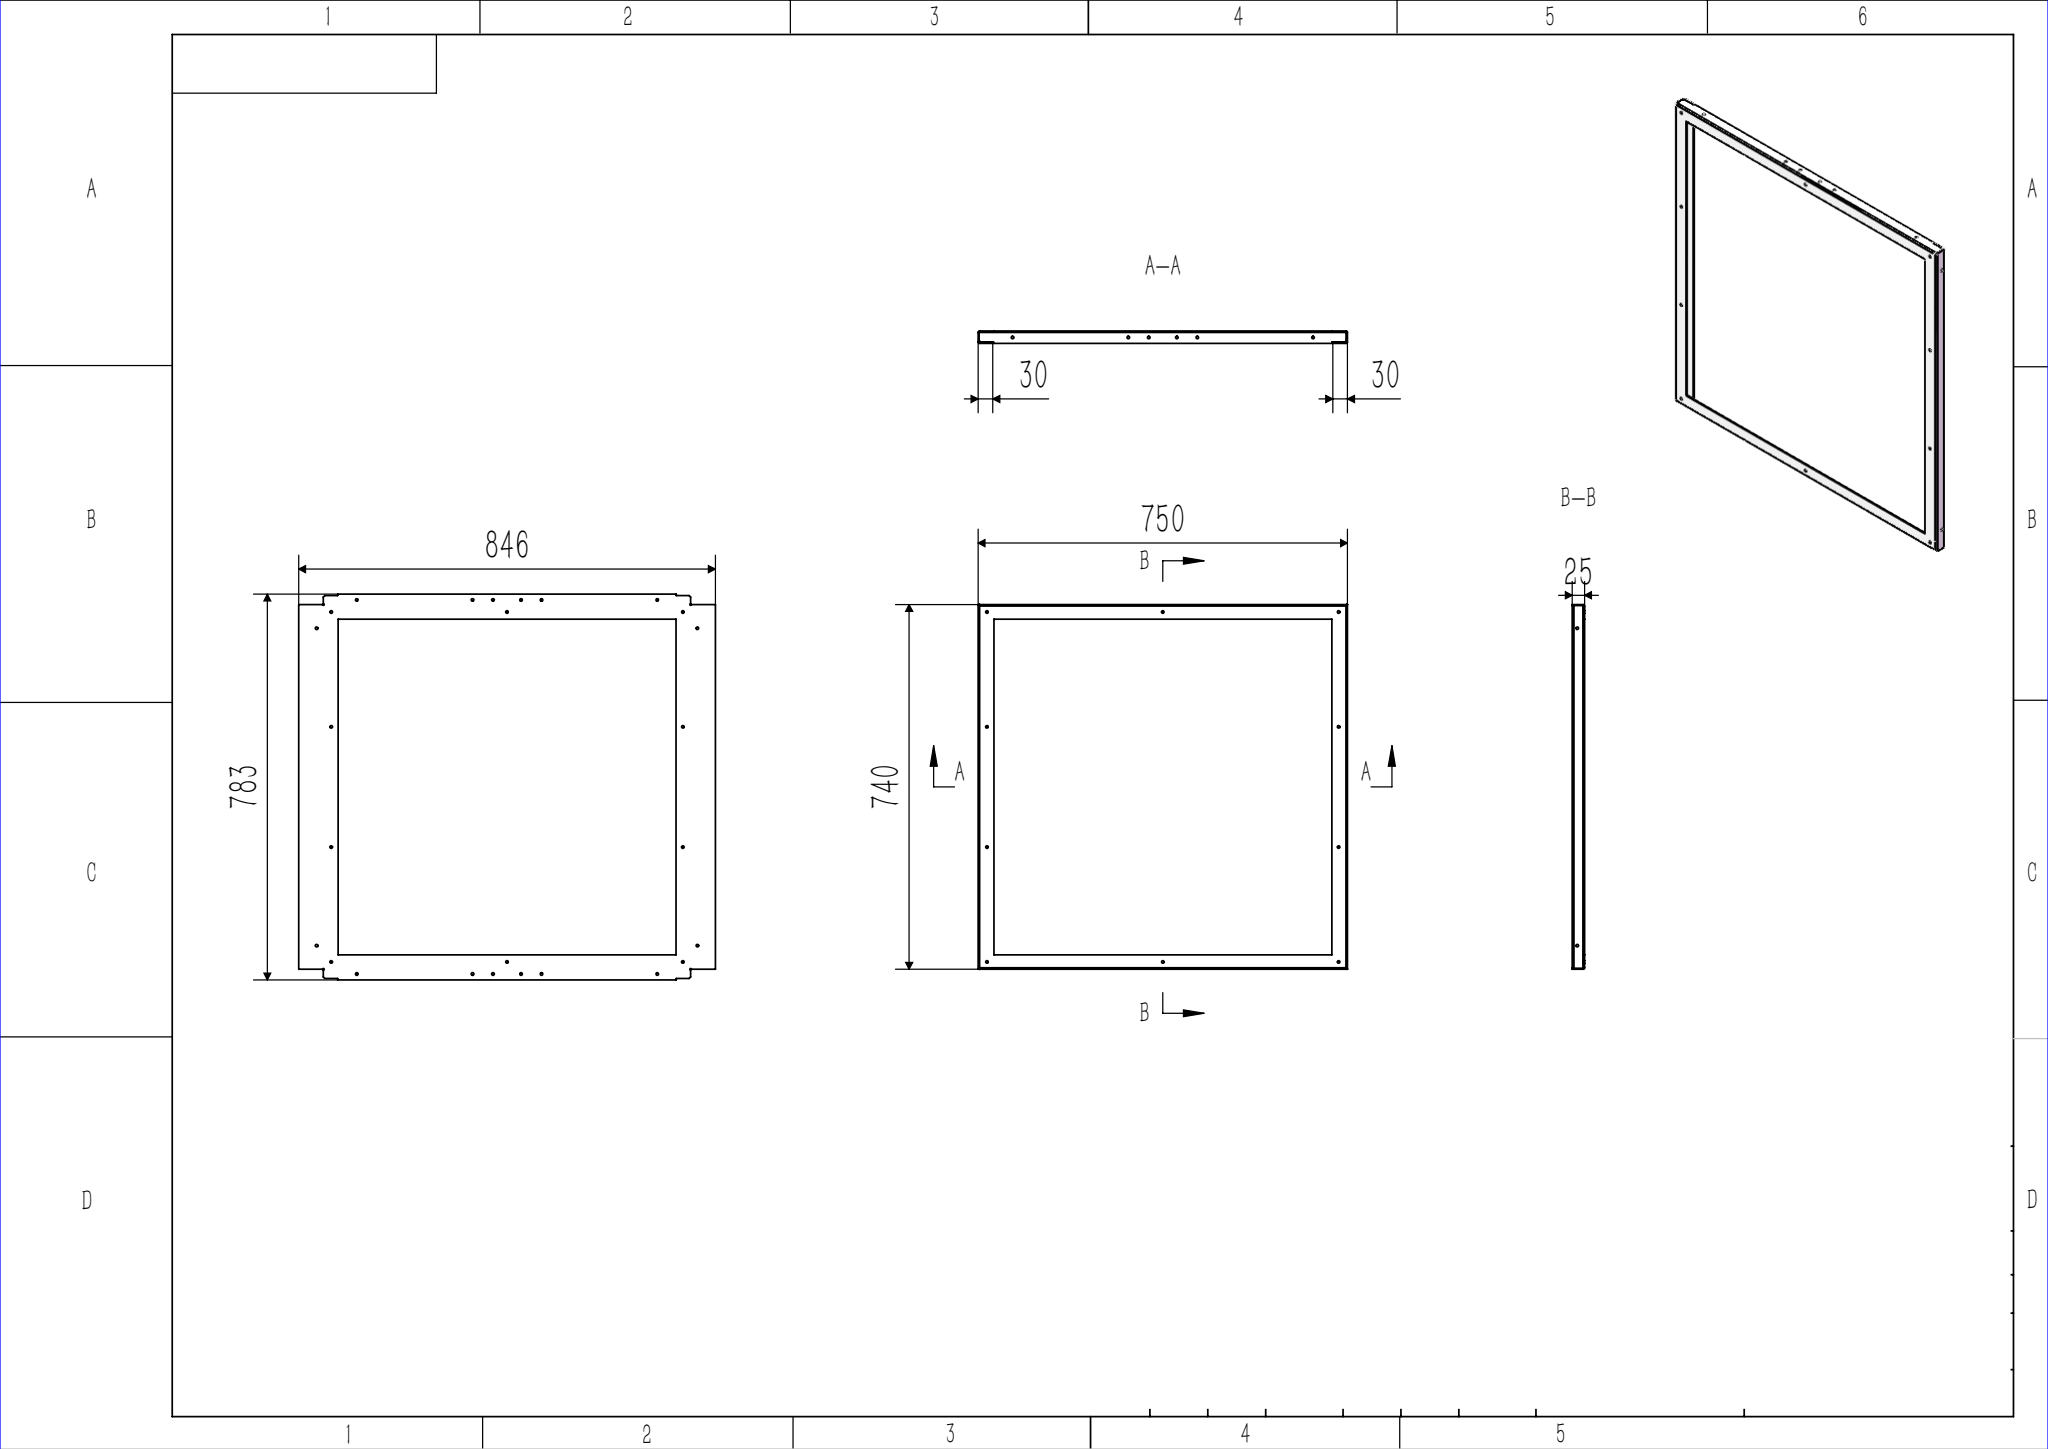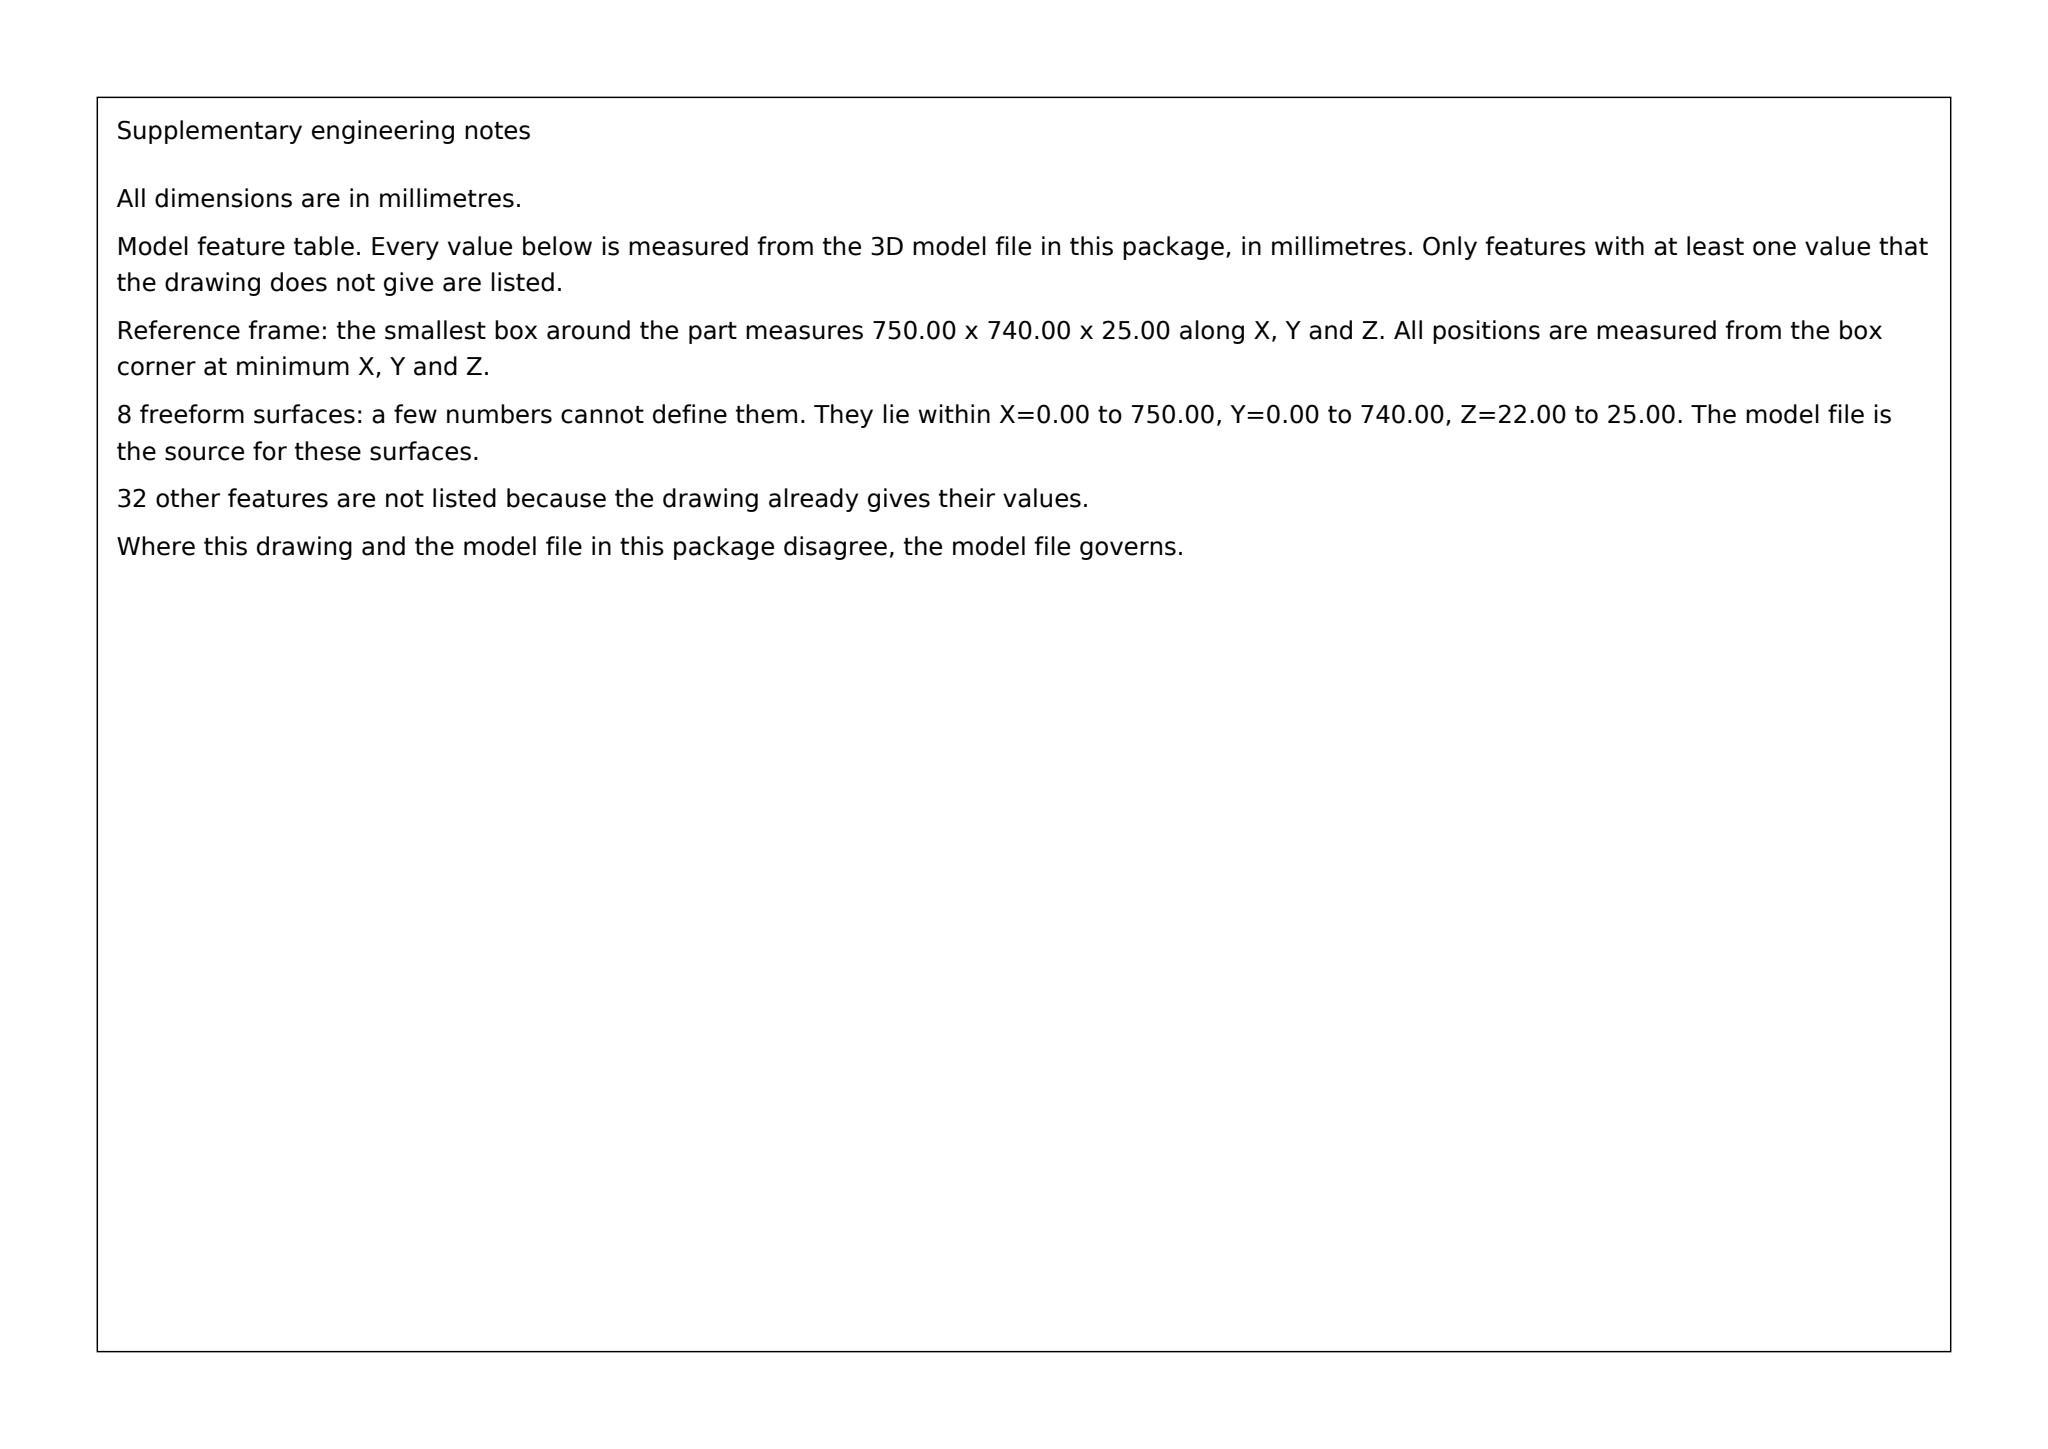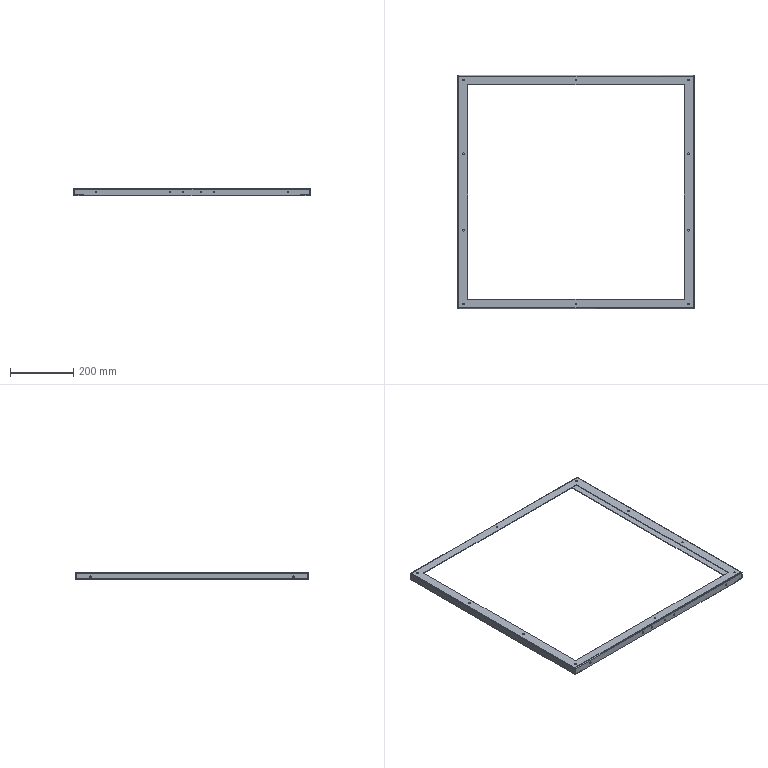Part | SolidWorks | mm | 1 solid | 122 faces | box 750 x 740 x 25 mm | volume 385716 mm3 | cylinder 64 | plane 50 | spline 8 | commonest cylinder face diameters 5.2 x52 2 x6 6 x6
Drawing notes:
SECT B-B: 26X Ø5.2 IN SIDE WALLS, C/L 10 FROM BACK FACE | from the solid: Ø5.2 x-axis holes at z=10.0 (y=48.02 & 692.02), 4 ea; part thk 25
SECT A-A: Ø5.2 IN TOP/BTM RAILS, C/L 12 FROM BACK FACE | from the solid: Ø5.2 y-axis holes at z=12.0 (x=70.02,305.02,346.52,403.52,445.02,680.02)
LH VIEW REF ONLY - TRUE ENVELOPE 750 X 740 X 25 | from the solid: bbox_xyz = 750.02 x 740.04 x 25.02
FACE HOLES Ø5.2 THRU: X=18, 375, 732; Y=15, 248, 492, 725 | from the solid: Ø5.2 z-axis holes at (18.02/375.02/732.02, 15.02/248.02/492.02/725.02)
ALL BENDS 90°, INSIDE R1; FLANGE 32 ON X SIDES, 29.5 ON Y SIDES | from the solid: x planes 0.02/2.02/30.02/32.02; y planes 0.02/2.02/29.52/710.52/738.02/740.02
A-A: 1ST RAIL Ø5.2 HOLE 70 FROM END FACE, TYP BOTH ENDS | from the solid: Ø5.2 y-axis holes at x=70.02 & 680.02 (bbox X=750.02); chain 70-235-41.5-57-41.5-235-70
FACE Ø5.2 PATTERN: 10X; NO HOLES AT X375/Y248 & X375/Y492 | from the solid: z-axis Ø5.2 holes only at (18,15)(18,248)(18,492)(18,725)(375,15)(375,725)(732,15)(732,248)(732,492)(732,725)